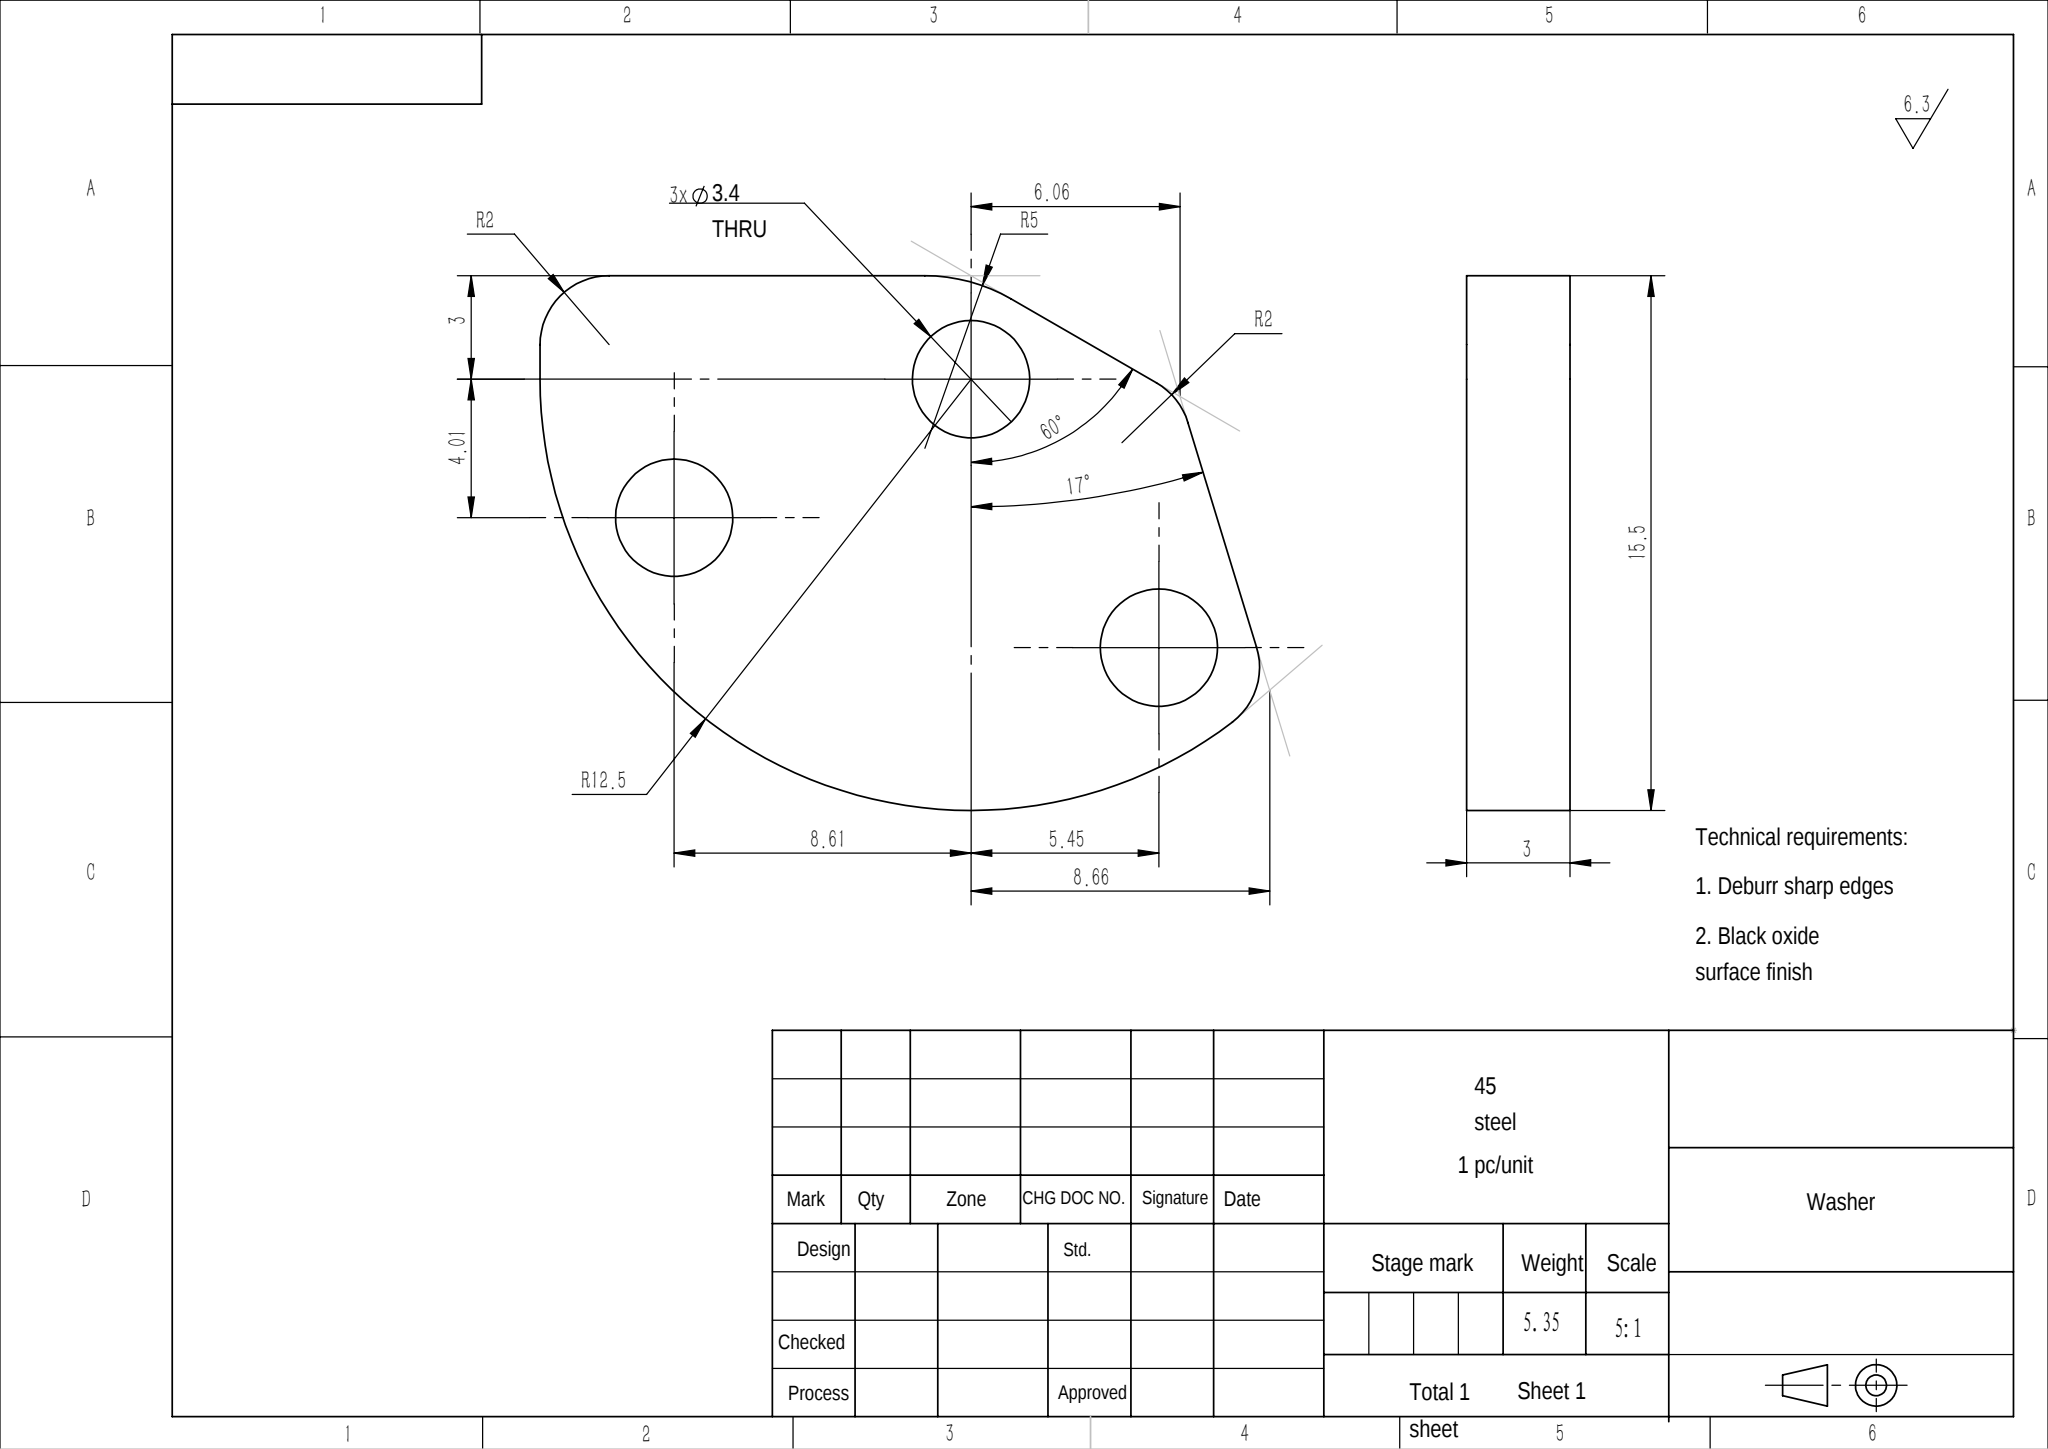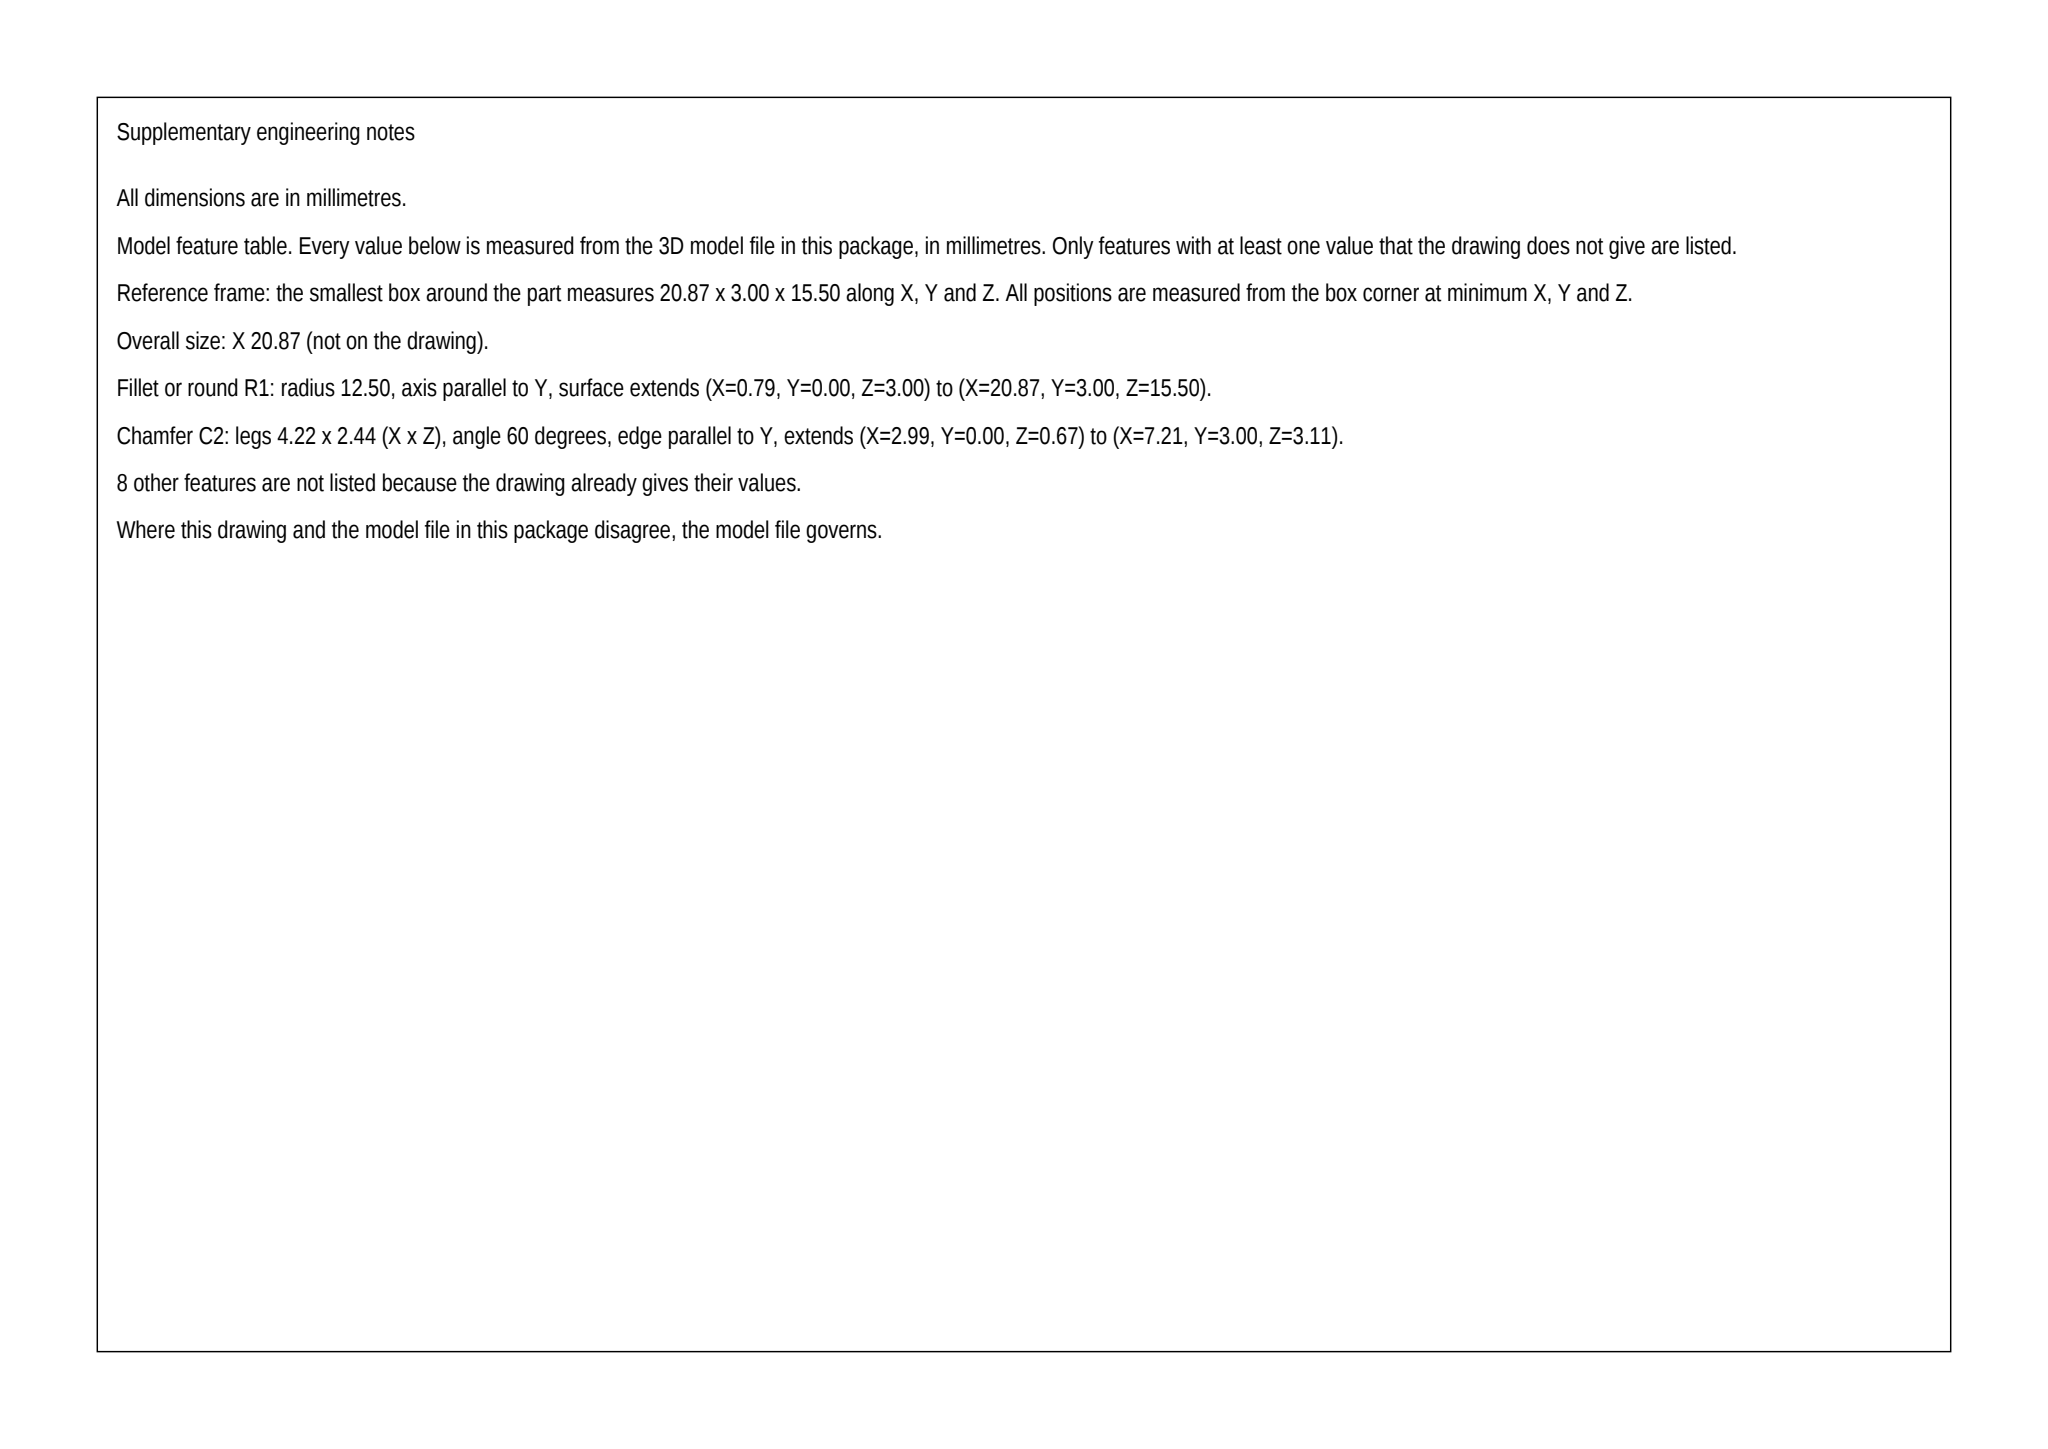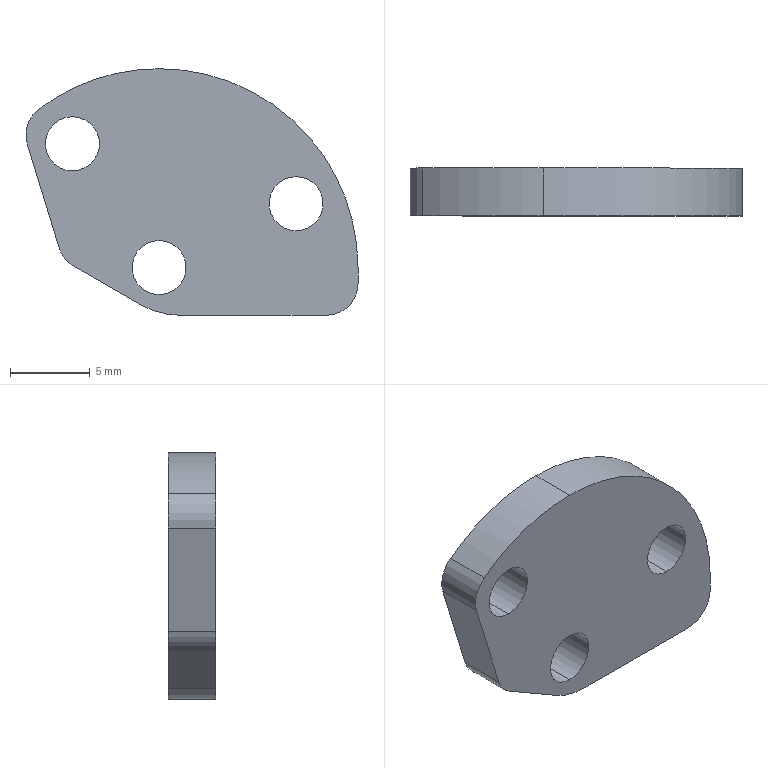Part | SolidWorks | mm | material 45 steel | 1 solid | 18 faces | box 20.87 x 3 x 15.5 mm | volume 677 mm3 | cylinder 12 | plane 6 | commonest cylinder face diameters 3.4 x6 4 x3 25 x2 10 x1
STEP:
#1=CARTESIAN_POINT('',(0.,3.,-0.2));
#2=VERTEX_POINT('',#1);
#3=CARTESIAN_POINT('',(0.,3.,3.2));
#4=VERTEX_POINT('',#3);
#5=CARTESIAN_POINT('',(0.,3.,1.5));
#6=DIRECTION('',(0.,1.,0.));
#7=DIRECTION('',(0.,0.,1.));
#8=AXIS2_PLACEMENT_3D('',#5,#6,#7);
#9=CIRCLE('',#8,1.7);
#10=EDGE_CURVE('',#2,#4,#9,.T.);
#11=ORIENTED_EDGE('',*,*,#10,.T.);
#12=CARTESIAN_POINT('',(0.,0.,3.2));
#13=VERTEX_POINT('',#12);
#14=CARTESIAN_POINT('',(0.,0.,3.2));
#15=DIRECTION('',(0.,-1.,0.));
#16=VECTOR('',#15,1000.);
#17=LINE('',#14,#16);
#18=EDGE_CURVE('',#4,#13,#17,.T.);
#19=ORIENTED_EDGE('',*,*,#18,.T.);
#20=CARTESIAN_POINT('',(0.,0.,-0.2));
#21=VERTEX_POINT('',#20);
#22=CARTESIAN_POINT('',(0.,0.,1.5));
#23=DIRECTION('',(0.,-1.,0.));
#24=DIRECTION('',(0.,0.,-1.));
#25=AXIS2_PLACEMENT_3D('',#22,#23,#24);
#26=CIRCLE('',#25,1.7);
#27=EDGE_CURVE('',#13,#21,#26,.T.);
#28=ORIENTED_EDGE('',*,*,#27,.T.);
#29=CARTESIAN_POINT('',(0.,0.,-0.2));
#30=DIRECTION('',(0.,-1.,0.));
#31=VECTOR('',#30,1000.);
#32=LINE('',#29,#31);
#33=EDGE_CURVE('',#2,#21,#32,.T.);
#34=ORIENTED_EDGE('',*,*,#33,.F.);
#35=EDGE_LOOP('',(#11,#19,#28,#34));
#36=FACE_OUTER_BOUND('',#35,.T.);
#37=CARTESIAN_POINT('',(0.,0.,1.5));
#38=DIRECTION('',(0.,-1.,0.));
#39=DIRECTION('',(0.,0.,-1.));
#40=AXIS2_PLACEMENT_3D('',#37,#38,#39);
#41=CYLINDRICAL_SURFACE('',#40,1.7);
#42=ADVANCED_FACE('',(#36),#41,.F.);
#43=CARTESIAN_POINT('',(8.61,3.,3.815));
#44=VERTEX_POINT('',#43);
#45=CARTESIAN_POINT('',(8.61,3.,7.215));
#46=VERTEX_POINT('',#45);
#47=CARTESIAN_POINT('',(8.61,3.,5.515));
#48=DIRECTION('',(0.,1.,0.));
#49=DIRECTION('',(0.,0.,1.));
#50=AXIS2_PLACEMENT_3D('',#47,#48,#49);
#51=CIRCLE('',#50,1.7);
#52=EDGE_CURVE('',#44,#46,#51,.T.);
#53=ORIENTED_EDGE('',*,*,#52,.T.);
#54=CARTESIAN_POINT('',(8.61,0.,7.215));
#55=VERTEX_POINT('',#54);
#56=CARTESIAN_POINT('',(8.61,0.,7.215));
#57=DIRECTION('',(0.,-1.,0.));
#58=VECTOR('',#57,1000.);
#59=LINE('',#56,#58);
#60=EDGE_CURVE('',#46,#55,#59,.T.);
#61=ORIENTED_EDGE('',*,*,#60,.T.);
#62=CARTESIAN_POINT('',(8.61,0.,3.815));
#63=VERTEX_POINT('',#62);
#64=CARTESIAN_POINT('',(8.61,0.,5.515));
#65=DIRECTION('',(0.,-1.,0.));
#66=DIRECTION('',(0.,0.,-1.));
#67=AXIS2_PLACEMENT_3D('',#64,#65,#66);
#68=CIRCLE('',#67,1.7);
#69=EDGE_CURVE('',#55,#63,#68,.T.);
#70=ORIENTED_EDGE('',*,*,#69,.T.);
#71=CARTESIAN_POINT('',(8.61,0.,3.815));
#72=DIRECTION('',(0.,-1.,0.));
#73=VECTOR('',#72,1000.);
#74=LINE('',#71,#73);
#75=EDGE_CURVE('',#44,#63,#74,.T.);
#76=ORIENTED_EDGE('',*,*,#75,.F.);
#77=EDGE_LOOP('',(#53,#61,#70,#76));
#78=FACE_OUTER_BOUND('',#77,.T.);
#79=CARTESIAN_POINT('',(8.61,0.,5.515));
#80=DIRECTION('',(0.,-1.,0.));
#81=DIRECTION('',(0.,0.,-1.));
#82=AXIS2_PLACEMENT_3D('',#79,#80,#81);
#83=CYLINDRICAL_SURFACE('',#82,1.7);
#84=ADVANCED_FACE('',(#78),#83,.F.);
#85=CARTESIAN_POINT('',(-5.449,3.,7.582));
#86=VERTEX_POINT('',#85);
#87=CARTESIAN_POINT('',(-5.449,3.,10.982));
#88=VERTEX_POINT('',#87);
#89=CARTESIAN_POINT('',(-5.449,3.,9.282));
#90=DIRECTION('',(0.,1.,0.));
#91=DIRECTION('',(0.,0.,1.));
#92=AXIS2_PLACEMENT_3D('',#89,#90,#91);
#93=CIRCLE('',#92,1.7);
#94=EDGE_CURVE('',#86,#88,#93,.T.);
#95=ORIENTED_EDGE('',*,*,#94,.T.);
#96=CARTESIAN_POINT('',(-5.449,0.,10.982));
#97=VERTEX_POINT('',#96);
#98=CARTESIAN_POINT('',(-5.449,0.,10.982));
#99=DIRECTION('',(0.,-1.,0.));
#100=VECTOR('',#99,1000.);
#101=LINE('',#98,#100);
#102=EDGE_CURVE('',#88,#97,#101,.T.);
#103=ORIENTED_EDGE('',*,*,#102,.T.);
#104=CARTESIAN_POINT('',(-5.449,0.,7.582));
#105=VERTEX_POINT('',#104);
#106=CARTESIAN_POINT('',(-5.449,0.,9.282));
#107=DIRECTION('',(0.,-1.,0.));
#108=DIRECTION('',(0.,0.,-1.));
#109=AXIS2_PLACEMENT_3D('',#106,#107,#108);
#110=CIRCLE('',#109,1.7);
#111=EDGE_CURVE('',#97,#105,#110,.T.);
#112=ORIENTED_EDGE('',*,*,#111,.T.);
#113=CARTESIAN_POINT('',(-5.449,0.,7.582));
#114=DIRECTION('',(0.,-1.,0.));
#115=VECTOR('',#114,1000.);
#116=LINE('',#113,#115);
#117=EDGE_CURVE('',#86,#105,#116,.T.);
#118=ORIENTED_EDGE('',*,*,#117,.F.);
#119=EDGE_LOOP('',(#95,#103,#112,#118));
#120=FACE_OUTER_BOUND('',#119,.T.);
#121=CARTESIAN_POINT('',(-5.449,0.,9.282));
#122=DIRECTION('',(0.,-1.,0.));
#123=DIRECTION('',(0.,0.,-1.));
#124=AXIS2_PLACEMENT_3D('',#121,#122,#123);
#125=CYLINDRICAL_SURFACE('',#124,1.7);
#126=ADVANCED_FACE('',(#120),#125,.F.);
#127=CARTESIAN_POINT('',(-7.582,0.,11.438));
#128=VERTEX_POINT('',#127);
#129=CARTESIAN_POINT('',(0.,0.,14.));
#130=VERTEX_POINT('',#129);
#131=CARTESIAN_POINT('',(0.,0.,1.5));
#132=DIRECTION('',(0.,1.,0.));
#133=DIRECTION('',(0.,0.,1.));
#134=AXIS2_PLACEMENT_3D('',#131,#132,#133);
#135=CIRCLE('',#134,12.5);
#136=EDGE_CURVE('',#128,#130,#135,.T.);
#137=ORIENTED_EDGE('',*,*,#136,.T.);
#138=CARTESIAN_POINT('',(0.,3.,14.));
#139=VERTEX_POINT('',#138);
#140=CARTESIAN_POINT('',(0.,0.,14.));
#141=DIRECTION('',(0.,1.,0.));
#142=VECTOR('',#141,1000.);
#143=LINE('',#140,#142);
#144=EDGE_CURVE('',#130,#139,#143,.T.);
#145=ORIENTED_EDGE('',*,*,#144,.T.);
#146=CARTESIAN_POINT('',(-7.582,3.,11.438));
#147=VERTEX_POINT('',#146);
#148=CARTESIAN_POINT('',(0.,3.,1.5));
#149=DIRECTION('',(0.,1.,0.));
#150=DIRECTION('',(0.,0.,1.));
#151=AXIS2_PLACEMENT_3D('',#148,#149,#150);
#152=CIRCLE('',#151,12.5);
#153=EDGE_CURVE('',#147,#139,#152,.T.);
#154=ORIENTED_EDGE('',*,*,#153,.F.);
#155=CARTESIAN_POINT('',(-7.582,0.,11.438));
#156=DIRECTION('',(0.,-1.,0.));
#157=VECTOR('',#156,1000.);
#158=LINE('',#155,#157);
#159=EDGE_CURVE('',#147,#128,#158,.T.);
#160=ORIENTED_EDGE('',*,*,#159,.T.);
#161=EDGE_LOOP('',(#137,#145,#154,#160));
#162=FACE_OUTER_BOUND('',#161,.T.);
#163=CARTESIAN_POINT('',(0.,0.,1.5));
#164=DIRECTION('',(0.,1.,0.));
#165=DIRECTION('',(0.,0.,1.));
#166=AXIS2_PLACEMENT_3D('',#163,#164,#165);
#167=CYLINDRICAL_SURFACE('',#166,12.5);
#168=ADVANCED_FACE('',(#162),#167,.T.);
#169=CARTESIAN_POINT('',(12.5,0.,1.5));
#170=VERTEX_POINT('',#169);
#171=CARTESIAN_POINT('',(12.5,0.,0.5));
#172=VERTEX_POINT('',#171);
#173=CARTESIAN_POINT('',(12.5,0.,-1.5));
#174=DIRECTION('',(-0.,0.,-1.));
#175=VECTOR('',#174,1000.);
#176=LINE('',#173,#175);
#177=EDGE_CURVE('',#170,#172,#176,.T.);
#178=ORIENTED_EDGE('',*,*,#177,.T.);
#179=CARTESIAN_POINT('',(12.5,3.,0.5));
#180=VERTEX_POINT('',#179);
#181=CARTESIAN_POINT('',(12.5,3.,0.5));
#182=DIRECTION('',(0.,1.,0.));
#183=VECTOR('',#182,1000.);
#184=LINE('',#181,#183);
#185=EDGE_CURVE('',#172,#180,#184,.T.);
#186=ORIENTED_EDGE('',*,*,#185,.T.);
#187=CARTESIAN_POINT('',(12.5,3.,1.5));
#188=VERTEX_POINT('',#187);
#189=CARTESIAN_POINT('',(12.5,3.,-1.5));
#190=DIRECTION('',(-0.,0.,-1.));
#191=VECTOR('',#190,1000.);
#192=LINE('',#189,#191);
#193=EDGE_CURVE('',#188,#180,#192,.T.);
#194=ORIENTED_EDGE('',*,*,#193,.F.);
#195=CARTESIAN_POINT('',(12.5,3.,1.5));
#196=DIRECTION('',(0.,-1.,0.));
#197=VECTOR('',#196,1000.);
#198=LINE('',#195,#197);
#199=EDGE_CURVE('',#188,#170,#198,.T.);
#200=ORIENTED_EDGE('',*,*,#199,.T.);
#201=EDGE_LOOP('',(#178,#186,#194,#200));
#202=FACE_OUTER_BOUND('',#201,.T.);
#203=CARTESIAN_POINT('',(12.5,3.,-1.5));
#204=DIRECTION('',(-1.,0.,0.));
#205=DIRECTION('',(0.,0.,1.));
#206=AXIS2_PLACEMENT_3D('',#203,#204,#205);
#207=PLANE('',#206);
#208=ADVANCED_FACE('',(#202),#207,.F.);
#209=CARTESIAN_POINT('',(10.5,0.,-1.5));
#210=VERTEX_POINT('',#209);
#211=CARTESIAN_POINT('',(1.34,0.,-1.5));
#212=VERTEX_POINT('',#211);
#213=CARTESIAN_POINT('',(-12.5,0.,-1.5));
#214=DIRECTION('',(-1.,0.,0.));
#215=VECTOR('',#214,1000.);
#216=LINE('',#213,#215);
#217=EDGE_CURVE('',#210,#212,#216,.T.);
#218=ORIENTED_EDGE('',*,*,#217,.T.);
#219=CARTESIAN_POINT('',(1.34,3.,-1.5));
#220=VERTEX_POINT('',#219);
#221=CARTESIAN_POINT('',(1.34,3.,-1.5));
#222=DIRECTION('',(0.,1.,0.));
#223=VECTOR('',#222,1000.);
#224=LINE('',#221,#223);
#225=EDGE_CURVE('',#212,#220,#224,.T.);
#226=ORIENTED_EDGE('',*,*,#225,.T.);
#227=CARTESIAN_POINT('',(10.5,3.,-1.5));
#228=VERTEX_POINT('',#227);
#229=CARTESIAN_POINT('',(-12.5,3.,-1.5));
#230=DIRECTION('',(-1.,0.,0.));
#231=VECTOR('',#230,1000.);
#232=LINE('',#229,#231);
#233=EDGE_CURVE('',#228,#220,#232,.T.);
#234=ORIENTED_EDGE('',*,*,#233,.F.);
#235=CARTESIAN_POINT('',(10.5,3.,-1.5));
#236=DIRECTION('',(0.,-1.,0.));
#237=VECTOR('',#236,1000.);
#238=LINE('',#235,#237);
#239=EDGE_CURVE('',#228,#210,#238,.T.);
#240=ORIENTED_EDGE('',*,*,#239,.T.);
#241=EDGE_LOOP('',(#218,#226,#234,#240));
#242=FACE_OUTER_BOUND('',#241,.T.);
#243=CARTESIAN_POINT('',(-12.5,3.,-1.5));
#244=DIRECTION('',(0.,0.,1.));
#245=DIRECTION('',(1.,0.,0.));
#246=AXIS2_PLACEMENT_3D('',#243,#244,#245);
#247=PLANE('',#246);
#248=ADVANCED_FACE('',(#242),#247,.F.);
#249=ORIENTED_EDGE('',*,*,#10,.F.);
#250=CARTESIAN_POINT('',(0.,3.,1.5));
#251=DIRECTION('',(0.,1.,0.));
#252=DIRECTION('',(0.,0.,1.));
#253=AXIS2_PLACEMENT_3D('',#250,#251,#252);
#254=CIRCLE('',#253,1.7);
#255=EDGE_CURVE('',#4,#2,#254,.T.);
#256=ORIENTED_EDGE('',*,*,#255,.F.);
#257=EDGE_LOOP('',(#249,#256));
#258=FACE_BOUND('',#257,.T.);
#259=ORIENTED_EDGE('',*,*,#52,.F.);
#260=CARTESIAN_POINT('',(8.61,3.,5.515));
#261=DIRECTION('',(0.,1.,0.));
#262=DIRECTION('',(0.,0.,1.));
#263=AXIS2_PLACEMENT_3D('',#260,#261,#262);
#264=CIRCLE('',#263,1.7);
#265=EDGE_CURVE('',#46,#44,#264,.T.);
#266=ORIENTED_EDGE('',*,*,#265,.F.);
#267=EDGE_LOOP('',(#259,#266));
#268=FACE_BOUND('',#267,.T.);
#269=ORIENTED_EDGE('',*,*,#94,.F.);
#270=CARTESIAN_POINT('',(-5.449,3.,9.282));
#271=DIRECTION('',(0.,1.,0.));
#272=DIRECTION('',(0.,0.,1.));
#273=AXIS2_PLACEMENT_3D('',#270,#271,#272);
#274=CIRCLE('',#273,1.7);
#275=EDGE_CURVE('',#88,#86,#274,.T.);
#276=ORIENTED_EDGE('',*,*,#275,.F.);
#277=EDGE_LOOP('',(#269,#276));
#278=FACE_BOUND('',#277,.T.);
#279=ORIENTED_EDGE('',*,*,#233,.T.);
#280=CARTESIAN_POINT('',(-1.16,3.,-0.8301));
#281=VERTEX_POINT('',#280);
#282=CARTESIAN_POINT('',(1.34,3.,3.5));
#283=DIRECTION('',(0.,1.,0.));
#284=DIRECTION('',(0.,0.,1.));
#285=AXIS2_PLACEMENT_3D('',#282,#283,#284);
#286=CIRCLE('',#285,5.);
#287=EDGE_CURVE('',#220,#281,#286,.T.);
#288=ORIENTED_EDGE('',*,*,#287,.T.);
#289=CARTESIAN_POINT('',(-5.379,3.,1.606));
#290=VERTEX_POINT('',#289);
#291=CARTESIAN_POINT('',(0.,3.,-1.5));
#292=DIRECTION('',(0.866,0.,-0.5));
#293=VECTOR('',#292,1000.);
#294=LINE('',#291,#293);
#295=EDGE_CURVE('',#290,#281,#294,.T.);
#296=ORIENTED_EDGE('',*,*,#295,.F.);
#297=CARTESIAN_POINT('',(-6.292,3.,2.753));
#298=VERTEX_POINT('',#297);
#299=CARTESIAN_POINT('',(-4.379,3.,3.338));
#300=DIRECTION('',(0.,1.,0.));
#301=DIRECTION('',(0.,0.,1.));
#302=AXIS2_PLACEMENT_3D('',#299,#300,#301);
#303=CIRCLE('',#302,2.);
#304=EDGE_CURVE('',#290,#298,#303,.T.);
#305=ORIENTED_EDGE('',*,*,#304,.T.);
#306=CARTESIAN_POINT('',(-8.282,3.,9.263));
#307=VERTEX_POINT('',#306);
#308=CARTESIAN_POINT('',(-4.985,3.,-1.524));
#309=DIRECTION('',(-0.2923,0.,0.9563));
#310=VECTOR('',#309,1000.);
#311=LINE('',#308,#310);
#312=EDGE_CURVE('',#298,#307,#311,.T.);
#313=ORIENTED_EDGE('',*,*,#312,.T.);
#314=CARTESIAN_POINT('',(-6.369,3.,9.848));
#315=DIRECTION('',(0.,1.,0.));
#316=DIRECTION('',(0.,0.,1.));
#317=AXIS2_PLACEMENT_3D('',#314,#315,#316);
#318=CIRCLE('',#317,2.);
#319=EDGE_CURVE('',#307,#147,#318,.T.);
#320=ORIENTED_EDGE('',*,*,#319,.T.);
#321=ORIENTED_EDGE('',*,*,#153,.T.);
#322=CARTESIAN_POINT('',(0.,3.,1.5));
#323=DIRECTION('',(0.,1.,0.));
#324=DIRECTION('',(0.,0.,1.));
#325=AXIS2_PLACEMENT_3D('',#322,#323,#324);
#326=CIRCLE('',#325,12.5);
#327=EDGE_CURVE('',#139,#188,#326,.T.);
#328=ORIENTED_EDGE('',*,*,#327,.T.);
#329=ORIENTED_EDGE('',*,*,#193,.T.);
#330=CARTESIAN_POINT('',(10.5,3.,0.5));
#331=DIRECTION('',(0.,1.,0.));
#332=DIRECTION('',(0.,0.,1.));
#333=AXIS2_PLACEMENT_3D('',#330,#331,#332);
#334=CIRCLE('',#333,2.);
#335=EDGE_CURVE('',#180,#228,#334,.T.);
#336=ORIENTED_EDGE('',*,*,#335,.T.);
#337=EDGE_LOOP('',(#279,#288,#296,#305,#313,#320,#321,#328,#329,#336));
#338=FACE_OUTER_BOUND('',#337,.T.);
#339=CARTESIAN_POINT('',(0.,3.,0.));
#340=DIRECTION('',(0.,1.,0.));
#341=DIRECTION('',(0.,0.,1.));
#342=AXIS2_PLACEMENT_3D('',#339,#340,#341);
#343=PLANE('',#342);
#344=ADVANCED_FACE('',(#258,#268,#278,#338),#343,.T.);
#345=CARTESIAN_POINT('',(0.,0.,1.5));
#346=DIRECTION('',(0.,-1.,0.));
#347=DIRECTION('',(0.,0.,-1.));
#348=AXIS2_PLACEMENT_3D('',#345,#346,#347);
#349=CIRCLE('',#348,1.7);
#350=EDGE_CURVE('',#21,#13,#349,.T.);
#351=ORIENTED_EDGE('',*,*,#350,.F.);
#352=ORIENTED_EDGE('',*,*,#27,.F.);
#353=EDGE_LOOP('',(#351,#352));
#354=FACE_BOUND('',#353,.T.);
#355=CARTESIAN_POINT('',(8.61,0.,5.515));
#356=DIRECTION('',(0.,-1.,0.));
#357=DIRECTION('',(0.,0.,-1.));
#358=AXIS2_PLACEMENT_3D('',#355,#356,#357);
#359=CIRCLE('',#358,1.7);
#360=EDGE_CURVE('',#63,#55,#359,.T.);
#361=ORIENTED_EDGE('',*,*,#360,.F.);
#362=ORIENTED_EDGE('',*,*,#69,.F.);
#363=EDGE_LOOP('',(#361,#362));
#364=FACE_BOUND('',#363,.T.);
#365=CARTESIAN_POINT('',(-5.449,0.,9.282));
#366=DIRECTION('',(0.,-1.,0.));
#367=DIRECTION('',(0.,0.,-1.));
#368=AXIS2_PLACEMENT_3D('',#365,#366,#367);
#369=CIRCLE('',#368,1.7);
#370=EDGE_CURVE('',#105,#97,#369,.T.);
#371=ORIENTED_EDGE('',*,*,#370,.F.);
#372=ORIENTED_EDGE('',*,*,#111,.F.);
#373=EDGE_LOOP('',(#371,#372));
#374=FACE_BOUND('',#373,.T.);
#375=CARTESIAN_POINT('',(-5.379,0.,1.606));
#376=VERTEX_POINT('',#375);
#377=CARTESIAN_POINT('',(-1.16,0.,-0.8301));
#378=VERTEX_POINT('',#377);
#379=CARTESIAN_POINT('',(0.,0.,-1.5));
#380=DIRECTION('',(0.866,0.,-0.5));
#381=VECTOR('',#380,1000.);
#382=LINE('',#379,#381);
#383=EDGE_CURVE('',#376,#378,#382,.T.);
#384=ORIENTED_EDGE('',*,*,#383,.T.);
#385=CARTESIAN_POINT('',(1.34,0.,3.5));
#386=DIRECTION('',(0.,-1.,0.));
#387=DIRECTION('',(0.,0.,1.));
#388=AXIS2_PLACEMENT_3D('',#385,#386,#387);
#389=CIRCLE('',#388,5.);
#390=EDGE_CURVE('',#378,#212,#389,.T.);
#391=ORIENTED_EDGE('',*,*,#390,.T.);
#392=ORIENTED_EDGE('',*,*,#217,.F.);
#393=CARTESIAN_POINT('',(10.5,0.,0.5));
#394=DIRECTION('',(0.,-1.,0.));
#395=DIRECTION('',(0.,0.,1.));
#396=AXIS2_PLACEMENT_3D('',#393,#394,#395);
#397=CIRCLE('',#396,2.);
#398=EDGE_CURVE('',#210,#172,#397,.T.);
#399=ORIENTED_EDGE('',*,*,#398,.T.);
#400=ORIENTED_EDGE('',*,*,#177,.F.);
#401=CARTESIAN_POINT('',(0.,0.,1.5));
#402=DIRECTION('',(0.,1.,0.));
#403=DIRECTION('',(0.,0.,1.));
#404=AXIS2_PLACEMENT_3D('',#401,#402,#403);
#405=CIRCLE('',#404,12.5);
#406=EDGE_CURVE('',#130,#170,#405,.T.);
#407=ORIENTED_EDGE('',*,*,#406,.F.);
#408=ORIENTED_EDGE('',*,*,#136,.F.);
#409=CARTESIAN_POINT('',(-8.282,0.,9.263));
#410=VERTEX_POINT('',#409);
#411=CARTESIAN_POINT('',(-6.369,0.,9.848));
#412=DIRECTION('',(0.,-1.,0.));
#413=DIRECTION('',(0.,0.,1.));
#414=AXIS2_PLACEMENT_3D('',#411,#412,#413);
#415=CIRCLE('',#414,2.);
#416=EDGE_CURVE('',#128,#410,#415,.T.);
#417=ORIENTED_EDGE('',*,*,#416,.T.);
#418=CARTESIAN_POINT('',(-6.292,0.,2.753));
#419=VERTEX_POINT('',#418);
#420=CARTESIAN_POINT('',(-6.062,0.,2.));
#421=DIRECTION('',(0.2923,0.,-0.9563));
#422=VECTOR('',#421,1000.);
#423=LINE('',#420,#422);
#424=EDGE_CURVE('',#410,#419,#423,.T.);
#425=ORIENTED_EDGE('',*,*,#424,.T.);
#426=CARTESIAN_POINT('',(-4.379,0.,3.338));
#427=DIRECTION('',(0.,-1.,0.));
#428=DIRECTION('',(0.,0.,1.));
#429=AXIS2_PLACEMENT_3D('',#426,#427,#428);
#430=CIRCLE('',#429,2.);
#431=EDGE_CURVE('',#419,#376,#430,.T.);
#432=ORIENTED_EDGE('',*,*,#431,.T.);
#433=EDGE_LOOP('',(#384,#391,#392,#399,#400,#407,#408,#417,#425,#432));
#434=FACE_OUTER_BOUND('',#433,.T.);
#435=CARTESIAN_POINT('',(0.,0.,0.));
#436=DIRECTION('',(0.,1.,0.));
#437=DIRECTION('',(0.,0.,1.));
#438=AXIS2_PLACEMENT_3D('',#435,#436,#437);
#439=PLANE('',#438);
#440=ADVANCED_FACE('',(#354,#364,#374,#434),#439,.F.);
#441=ORIENTED_EDGE('',*,*,#144,.F.);
#442=ORIENTED_EDGE('',*,*,#406,.T.);
#443=ORIENTED_EDGE('',*,*,#199,.F.);
#444=ORIENTED_EDGE('',*,*,#327,.F.);
#445=EDGE_LOOP('',(#441,#442,#443,#444));
#446=FACE_OUTER_BOUND('',#445,.T.);
#447=CARTESIAN_POINT('',(0.,0.,1.5));
#448=DIRECTION('',(0.,1.,0.));
#449=DIRECTION('',(0.,0.,1.));
#450=AXIS2_PLACEMENT_3D('',#447,#448,#449);
#451=CYLINDRICAL_SURFACE('',#450,12.5);
#452=ADVANCED_FACE('',(#446),#451,.T.);
#453=ORIENTED_EDGE('',*,*,#295,.T.);
#454=CARTESIAN_POINT('',(-1.16,0.,-0.8301));
#455=DIRECTION('',(0.,-1.,0.));
#456=VECTOR('',#455,1000.);
#457=LINE('',#454,#456);
#458=EDGE_CURVE('',#281,#378,#457,.T.);
#459=ORIENTED_EDGE('',*,*,#458,.T.);
#460=ORIENTED_EDGE('',*,*,#383,.F.);
#461=CARTESIAN_POINT('',(-5.379,3.,1.606));
#462=DIRECTION('',(0.,1.,0.));
#463=VECTOR('',#462,1000.);
#464=LINE('',#461,#463);
#465=EDGE_CURVE('',#376,#290,#464,.T.);
#466=ORIENTED_EDGE('',*,*,#465,.T.);
#467=EDGE_LOOP('',(#453,#459,#460,#466));
#468=FACE_OUTER_BOUND('',#467,.T.);
#469=CARTESIAN_POINT('',(0.,0.,-1.5));
#470=DIRECTION('',(0.5,0.,0.866));
#471=DIRECTION('',(0.866,0.,-0.5));
#472=AXIS2_PLACEMENT_3D('',#469,#470,#471);
#473=PLANE('',#472);
#474=ADVANCED_FACE('',(#468),#473,.F.);
#475=ORIENTED_EDGE('',*,*,#424,.F.);
#476=CARTESIAN_POINT('',(-8.282,0.,9.263));
#477=DIRECTION('',(0.,1.,0.));
#478=VECTOR('',#477,1000.);
#479=LINE('',#476,#478);
#480=EDGE_CURVE('',#410,#307,#479,.T.);
#481=ORIENTED_EDGE('',*,*,#480,.T.);
#482=ORIENTED_EDGE('',*,*,#312,.F.);
#483=CARTESIAN_POINT('',(-6.292,0.,2.753));
#484=DIRECTION('',(0.,-1.,0.));
#485=VECTOR('',#484,1000.);
#486=LINE('',#483,#485);
#487=EDGE_CURVE('',#298,#419,#486,.T.);
#488=ORIENTED_EDGE('',*,*,#487,.T.);
#489=EDGE_LOOP('',(#475,#481,#482,#488));
#490=FACE_OUTER_BOUND('',#489,.T.);
#491=CARTESIAN_POINT('',(-6.062,0.,2.));
#492=DIRECTION('',(0.9563,0.,0.2923));
#493=DIRECTION('',(0.,1.,0.));
#494=AXIS2_PLACEMENT_3D('',#491,#492,#493);
#495=PLANE('',#494);
#496=ADVANCED_FACE('',(#490),#495,.F.);
#497=ORIENTED_EDGE('',*,*,#102,.F.);
#498=ORIENTED_EDGE('',*,*,#275,.T.);
#499=ORIENTED_EDGE('',*,*,#117,.T.);
#500=ORIENTED_EDGE('',*,*,#370,.T.);
#501=EDGE_LOOP('',(#497,#498,#499,#500));
#502=FACE_OUTER_BOUND('',#501,.T.);
#503=CARTESIAN_POINT('',(-5.449,0.,9.282));
#504=DIRECTION('',(0.,-1.,0.));
#505=DIRECTION('',(0.,0.,-1.));
#506=AXIS2_PLACEMENT_3D('',#503,#504,#505);
#507=CYLINDRICAL_SURFACE('',#506,1.7);
#508=ADVANCED_FACE('',(#502),#507,.F.);
#509=ORIENTED_EDGE('',*,*,#60,.F.);
#510=ORIENTED_EDGE('',*,*,#265,.T.);
#511=ORIENTED_EDGE('',*,*,#75,.T.);
#512=ORIENTED_EDGE('',*,*,#360,.T.);
#513=EDGE_LOOP('',(#509,#510,#511,#512));
#514=FACE_OUTER_BOUND('',#513,.T.);
#515=CARTESIAN_POINT('',(8.61,0.,5.515));
#516=DIRECTION('',(0.,-1.,0.));
#517=DIRECTION('',(0.,0.,-1.));
#518=AXIS2_PLACEMENT_3D('',#515,#516,#517);
#519=CYLINDRICAL_SURFACE('',#518,1.7);
#520=ADVANCED_FACE('',(#514),#519,.F.);
#521=ORIENTED_EDGE('',*,*,#335,.F.);
#522=ORIENTED_EDGE('',*,*,#185,.F.);
#523=ORIENTED_EDGE('',*,*,#398,.F.);
#524=ORIENTED_EDGE('',*,*,#239,.F.);
#525=EDGE_LOOP('',(#521,#522,#523,#524));
#526=FACE_OUTER_BOUND('',#525,.T.);
#527=CARTESIAN_POINT('',(10.5,3.,0.5));
#528=DIRECTION('',(0.,-1.,0.));
#529=DIRECTION('',(0.,0.,-1.));
#530=AXIS2_PLACEMENT_3D('',#527,#528,#529);
#531=CYLINDRICAL_SURFACE('',#530,2.);
#532=ADVANCED_FACE('',(#526),#531,.T.);
#533=ORIENTED_EDGE('',*,*,#319,.F.);
#534=ORIENTED_EDGE('',*,*,#480,.F.);
#535=ORIENTED_EDGE('',*,*,#416,.F.);
#536=ORIENTED_EDGE('',*,*,#159,.F.);
#537=EDGE_LOOP('',(#533,#534,#535,#536));
#538=FACE_OUTER_BOUND('',#537,.T.);
#539=CARTESIAN_POINT('',(-6.369,0.,9.848));
#540=DIRECTION('',(0.,1.,0.));
#541=DIRECTION('',(0.,0.,1.));
#542=AXIS2_PLACEMENT_3D('',#539,#540,#541);
#543=CYLINDRICAL_SURFACE('',#542,2.);
#544=ADVANCED_FACE('',(#538),#543,.T.);
#545=ORIENTED_EDGE('',*,*,#431,.F.);
#546=ORIENTED_EDGE('',*,*,#487,.F.);
#547=ORIENTED_EDGE('',*,*,#304,.F.);
#548=ORIENTED_EDGE('',*,*,#465,.F.);
#549=EDGE_LOOP('',(#545,#546,#547,#548));
#550=FACE_OUTER_BOUND('',#549,.T.);
#551=CARTESIAN_POINT('',(-4.379,0.,3.338));
#552=DIRECTION('',(0.,1.,0.));
#553=DIRECTION('',(0.,0.,1.));
#554=AXIS2_PLACEMENT_3D('',#551,#552,#553);
#555=CYLINDRICAL_SURFACE('',#554,2.);
#556=ADVANCED_FACE('',(#550),#555,.T.);
#557=ORIENTED_EDGE('',*,*,#390,.F.);
#558=ORIENTED_EDGE('',*,*,#458,.F.);
#559=ORIENTED_EDGE('',*,*,#287,.F.);
#560=ORIENTED_EDGE('',*,*,#225,.F.);
#561=EDGE_LOOP('',(#557,#558,#559,#560));
#562=FACE_OUTER_BOUND('',#561,.T.);
#563=CARTESIAN_POINT('',(1.34,3.,3.5));
#564=DIRECTION('',(0.,1.,0.));
#565=DIRECTION('',(0.,0.,1.));
#566=AXIS2_PLACEMENT_3D('',#563,#564,#565);
#567=CYLINDRICAL_SURFACE('',#566,5.);
#568=ADVANCED_FACE('',(#562),#567,.T.);
#569=ORIENTED_EDGE('',*,*,#18,.F.);
#570=ORIENTED_EDGE('',*,*,#255,.T.);
#571=ORIENTED_EDGE('',*,*,#33,.T.);
#572=ORIENTED_EDGE('',*,*,#350,.T.);
#573=EDGE_LOOP('',(#569,#570,#571,#572));
#574=FACE_OUTER_BOUND('',#573,.T.);
#575=CARTESIAN_POINT('',(0.,0.,1.5));
#576=DIRECTION('',(0.,-1.,0.));
#577=DIRECTION('',(0.,0.,-1.));
#578=AXIS2_PLACEMENT_3D('',#575,#576,#577);
#579=CYLINDRICAL_SURFACE('',#578,1.7);
#580=ADVANCED_FACE('',(#574),#579,.F.);
#581=CLOSED_SHELL('',(#42,#84,#126,#168,#208,#248,#344,#440,#452,#474,#496,#508,#520,#532,#544,#556,#568,#580));
#582=MANIFOLD_SOLID_BREP('',#581);
#583=CARTESIAN_POINT('',(0.,0.,0.));
#584=DIRECTION('',(0.,0.,1.));
#585=DIRECTION('',(1.,0.,0.));
#586=AXIS2_PLACEMENT_3D('',#583,#584,#585);
#587=(LENGTH_UNIT()NAMED_UNIT(*)SI_UNIT(.MILLI.,.METRE.));
#588=UNCERTAINTY_MEASURE_WITH_UNIT(LENGTH_MEASURE(0.00001),#587,'','');
#589=(NAMED_UNIT(*)PLANE_ANGLE_UNIT()SI_UNIT($,.RADIAN.));
#590=(NAMED_UNIT(*)SI_UNIT($,.STERADIAN.)SOLID_ANGLE_UNIT());
#591=(GEOMETRIC_REPRESENTATION_CONTEXT(3)GLOBAL_UNCERTAINTY_ASSIGNED_CONTEXT((#588))GLOBAL_UNIT_ASSIGNED_CONTEXT((#587,#589,#590))REPRESENTATION_CONTEXT('',''));
#592=ADVANCED_BREP_SHAPE_REPRESENTATION('',(#582,#586),#591);